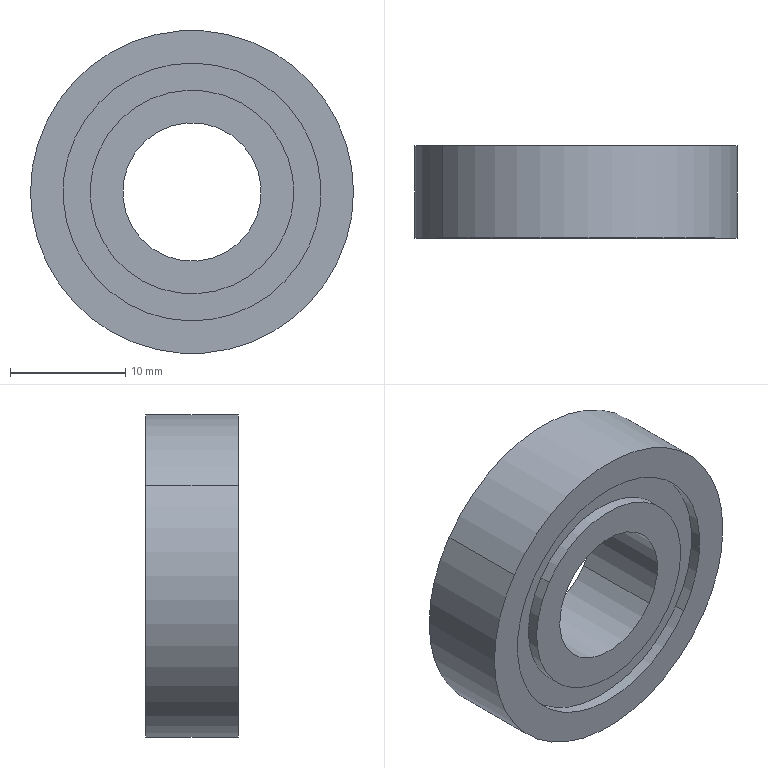Component | SolidWorks | UpperAxis-1_UpperSlideBearing-1 | 1 solid | 18 faces | box 28 x 8 x 28 mm | volume 3727 mm3 | cylinder 12 | plane 6 | commonest cylinder face diameters 17.655 x4 22.345 x4 28 x2 12 x2
build123d program:
from build123d import *


with BuildPart() as part:
    # Sketch1 → Revolve1 (revolve)
    with BuildSketch(Plane(origin=(0, 0, 0), x_dir=(1, 0, 0), z_dir=(0, 1, 0)), mode=Mode.PRIVATE) as revolve1_sk:
        Polygon((4, 4), (6.827, 4), (6.827, 3), (9.173, 3), (9.173, 4), (12, 4), (12, -4), (9.173, -4), (9.173, -3), (6.827, -3), (6.827, -4), (4, -4), align=None)
    revolve(revolve1_sk.sketch.rotate(Axis((-2, 0, -4.4), (0, 0, 1)), 180), axis=Axis((-2, 0, -4.4), (0, 0, 1)))


solid = part.part

# Placed as in the assembly
solid = solid.moved(Location((-776.65, 378.568, -31.569), (90, 0, 0)))
STEP:
#1=COLOUR_RGB('',0.7922,0.8196,0.9333);
#2=FILL_AREA_STYLE_COLOUR('',#1);
#3=FILL_AREA_STYLE('',(#2));
#4=SURFACE_STYLE_FILL_AREA(#3);
#5=SURFACE_SIDE_STYLE('',(#4));
#6=SURFACE_STYLE_USAGE(.BOTH.,#5);
#7=PRESENTATION_STYLE_ASSIGNMENT((#6));
#8=CARTESIAN_POINT('',(-30.943,14.747,-1.047));
#9=VERTEX_POINT('',#8);
#10=CARTESIAN_POINT('',(-30.368,14.747,-1.439));
#11=VERTEX_POINT('',#10);
#12=CARTESIAN_POINT('',(-30.655,14.747,-1.243));
#13=DIRECTION('',(-0.,1.,0.));
#14=DIRECTION('',(-0.8265,0.,0.563));
#15=AXIS2_PLACEMENT_3D('',#12,#13,#14);
#16=CIRCLE('',#15,0.3475);
#17=EDGE_CURVE('',#9,#11,#16,.T.);
#18=ORIENTED_EDGE('',*,*,#17,.T.);
#19=CARTESIAN_POINT('',(-30.368,14.786,-1.439));
#20=VERTEX_POINT('',#19);
#21=CARTESIAN_POINT('',(-30.368,15.077,-1.439));
#22=DIRECTION('',(-0.,1.,0.));
#23=VECTOR('',#22,39.37);
#24=LINE('',#21,#23);
#25=EDGE_CURVE('',#11,#20,#24,.T.);
#26=ORIENTED_EDGE('',*,*,#25,.T.);
#27=CARTESIAN_POINT('',(-30.943,14.786,-1.047));
#28=VERTEX_POINT('',#27);
#29=CARTESIAN_POINT('',(-30.655,14.786,-1.243));
#30=DIRECTION('',(-0.,1.,0.));
#31=DIRECTION('',(-0.8265,0.,0.563));
#32=AXIS2_PLACEMENT_3D('',#29,#30,#31);
#33=CIRCLE('',#32,0.3475);
#34=EDGE_CURVE('',#28,#20,#33,.T.);
#35=ORIENTED_EDGE('',*,*,#34,.F.);
#36=CARTESIAN_POINT('',(-30.943,15.077,-1.047));
#37=DIRECTION('',(-0.,1.,0.));
#38=VECTOR('',#37,39.37);
#39=LINE('',#36,#38);
#40=EDGE_CURVE('',#9,#28,#39,.T.);
#41=ORIENTED_EDGE('',*,*,#40,.F.);
#42=EDGE_LOOP('',(#18,#26,#35,#41));
#43=FACE_OUTER_BOUND('',#42,.T.);
#44=CARTESIAN_POINT('',(-30.655,15.077,-1.243));
#45=DIRECTION('',(-0.,1.,0.));
#46=DIRECTION('',(-0.8265,0.,0.563));
#47=AXIS2_PLACEMENT_3D('',#44,#45,#46);
#48=CYLINDRICAL_SURFACE('',#47,0.3475);
#49=ADVANCED_FACE('',(#43),#48,.T.);
#50=CARTESIAN_POINT('',(-30.292,14.747,-1.491));
#51=VERTEX_POINT('',#50);
#52=CARTESIAN_POINT('',(-31.019,14.747,-0.9953));
#53=VERTEX_POINT('',#52);
#54=CARTESIAN_POINT('',(-30.655,14.747,-1.243));
#55=DIRECTION('',(-0.,1.,0.));
#56=DIRECTION('',(-0.8265,0.,0.563));
#57=AXIS2_PLACEMENT_3D('',#54,#55,#56);
#58=CIRCLE('',#57,0.4399);
#59=EDGE_CURVE('',#51,#53,#58,.T.);
#60=ORIENTED_EDGE('',*,*,#59,.F.);
#61=CARTESIAN_POINT('',(-30.292,14.786,-1.491));
#62=VERTEX_POINT('',#61);
#63=CARTESIAN_POINT('',(-30.292,15.077,-1.491));
#64=DIRECTION('',(-0.,1.,0.));
#65=VECTOR('',#64,39.37);
#66=LINE('',#63,#65);
#67=EDGE_CURVE('',#51,#62,#66,.T.);
#68=ORIENTED_EDGE('',*,*,#67,.T.);
#69=CARTESIAN_POINT('',(-31.019,14.786,-0.9953));
#70=VERTEX_POINT('',#69);
#71=CARTESIAN_POINT('',(-30.655,14.786,-1.243));
#72=DIRECTION('',(-0.,1.,0.));
#73=DIRECTION('',(-0.8265,0.,0.563));
#74=AXIS2_PLACEMENT_3D('',#71,#72,#73);
#75=CIRCLE('',#74,0.4399);
#76=EDGE_CURVE('',#62,#70,#75,.T.);
#77=ORIENTED_EDGE('',*,*,#76,.T.);
#78=CARTESIAN_POINT('',(-31.019,15.077,-0.9953));
#79=DIRECTION('',(-0.,1.,0.));
#80=VECTOR('',#79,39.37);
#81=LINE('',#78,#80);
#82=EDGE_CURVE('',#53,#70,#81,.T.);
#83=ORIENTED_EDGE('',*,*,#82,.F.);
#84=EDGE_LOOP('',(#60,#68,#77,#83));
#85=FACE_OUTER_BOUND('',#84,.T.);
#86=CARTESIAN_POINT('',(-30.655,15.077,-1.243));
#87=DIRECTION('',(-0.,1.,0.));
#88=DIRECTION('',(-0.8265,0.,0.563));
#89=AXIS2_PLACEMENT_3D('',#86,#87,#88);
#90=CYLINDRICAL_SURFACE('',#89,0.4399);
#91=ADVANCED_FACE('',(#85),#90,.F.);
#92=CARTESIAN_POINT('',(-31.111,14.747,-0.9326));
#93=VERTEX_POINT('',#92);
#94=CARTESIAN_POINT('',(-30.2,14.747,-1.553));
#95=VERTEX_POINT('',#94);
#96=CARTESIAN_POINT('',(-30.655,14.747,-1.243));
#97=DIRECTION('',(-0.,1.,0.));
#98=DIRECTION('',(-0.8265,0.,0.563));
#99=AXIS2_PLACEMENT_3D('',#96,#97,#98);
#100=CIRCLE('',#99,0.5512);
#101=EDGE_CURVE('',#93,#95,#100,.T.);
#102=ORIENTED_EDGE('',*,*,#101,.T.);
#103=CARTESIAN_POINT('',(-30.2,15.062,-1.553));
#104=VERTEX_POINT('',#103);
#105=CARTESIAN_POINT('',(-30.2,15.077,-1.553));
#106=DIRECTION('',(-0.,1.,0.));
#107=VECTOR('',#106,39.37);
#108=LINE('',#105,#107);
#109=EDGE_CURVE('',#95,#104,#108,.T.);
#110=ORIENTED_EDGE('',*,*,#109,.T.);
#111=CARTESIAN_POINT('',(-31.111,15.062,-0.9326));
#112=VERTEX_POINT('',#111);
#113=CARTESIAN_POINT('',(-30.655,15.062,-1.243));
#114=DIRECTION('',(-0.,1.,0.));
#115=DIRECTION('',(-0.8265,0.,0.563));
#116=AXIS2_PLACEMENT_3D('',#113,#114,#115);
#117=CIRCLE('',#116,0.5512);
#118=EDGE_CURVE('',#112,#104,#117,.T.);
#119=ORIENTED_EDGE('',*,*,#118,.F.);
#120=CARTESIAN_POINT('',(-31.111,15.077,-0.9326));
#121=DIRECTION('',(-0.,1.,0.));
#122=VECTOR('',#121,39.37);
#123=LINE('',#120,#122);
#124=EDGE_CURVE('',#93,#112,#123,.T.);
#125=ORIENTED_EDGE('',*,*,#124,.F.);
#126=EDGE_LOOP('',(#102,#110,#119,#125));
#127=FACE_OUTER_BOUND('',#126,.T.);
#128=CARTESIAN_POINT('',(-30.655,15.077,-1.243));
#129=DIRECTION('',(-0.,1.,0.));
#130=DIRECTION('',(-0.8265,0.,0.563));
#131=AXIS2_PLACEMENT_3D('',#128,#129,#130);
#132=CYLINDRICAL_SURFACE('',#131,0.5512);
#133=ADVANCED_FACE('',(#127),#132,.T.);
#134=CARTESIAN_POINT('',(-30.292,15.022,-1.491));
#135=VERTEX_POINT('',#134);
#136=CARTESIAN_POINT('',(-31.019,15.022,-0.9953));
#137=VERTEX_POINT('',#136);
#138=CARTESIAN_POINT('',(-30.655,15.022,-1.243));
#139=DIRECTION('',(-0.,1.,0.));
#140=DIRECTION('',(-0.8265,0.,0.563));
#141=AXIS2_PLACEMENT_3D('',#138,#139,#140);
#142=CIRCLE('',#141,0.4399);
#143=EDGE_CURVE('',#135,#137,#142,.T.);
#144=ORIENTED_EDGE('',*,*,#143,.F.);
#145=CARTESIAN_POINT('',(-30.292,15.062,-1.491));
#146=VERTEX_POINT('',#145);
#147=CARTESIAN_POINT('',(-30.292,15.077,-1.491));
#148=DIRECTION('',(-0.,1.,0.));
#149=VECTOR('',#148,39.37);
#150=LINE('',#147,#149);
#151=EDGE_CURVE('',#135,#146,#150,.T.);
#152=ORIENTED_EDGE('',*,*,#151,.T.);
#153=CARTESIAN_POINT('',(-31.019,15.062,-0.9953));
#154=VERTEX_POINT('',#153);
#155=CARTESIAN_POINT('',(-30.655,15.062,-1.243));
#156=DIRECTION('',(-0.,1.,0.));
#157=DIRECTION('',(-0.8265,0.,0.563));
#158=AXIS2_PLACEMENT_3D('',#155,#156,#157);
#159=CIRCLE('',#158,0.4399);
#160=EDGE_CURVE('',#146,#154,#159,.T.);
#161=ORIENTED_EDGE('',*,*,#160,.T.);
#162=CARTESIAN_POINT('',(-31.019,15.077,-0.9953));
#163=DIRECTION('',(-0.,1.,0.));
#164=VECTOR('',#163,39.37);
#165=LINE('',#162,#164);
#166=EDGE_CURVE('',#137,#154,#165,.T.);
#167=ORIENTED_EDGE('',*,*,#166,.F.);
#168=EDGE_LOOP('',(#144,#152,#161,#167));
#169=FACE_OUTER_BOUND('',#168,.T.);
#170=CARTESIAN_POINT('',(-30.655,15.077,-1.243));
#171=DIRECTION('',(-0.,1.,0.));
#172=DIRECTION('',(-0.8265,0.,0.563));
#173=AXIS2_PLACEMENT_3D('',#170,#171,#172);
#174=CYLINDRICAL_SURFACE('',#173,0.4399);
#175=ADVANCED_FACE('',(#169),#174,.F.);
#176=CARTESIAN_POINT('',(-30.943,15.022,-1.047));
#177=VERTEX_POINT('',#176);
#178=CARTESIAN_POINT('',(-30.368,15.022,-1.439));
#179=VERTEX_POINT('',#178);
#180=CARTESIAN_POINT('',(-30.655,15.022,-1.243));
#181=DIRECTION('',(-0.,1.,0.));
#182=DIRECTION('',(-0.8265,0.,0.563));
#183=AXIS2_PLACEMENT_3D('',#180,#181,#182);
#184=CIRCLE('',#183,0.3475);
#185=EDGE_CURVE('',#177,#179,#184,.T.);
#186=ORIENTED_EDGE('',*,*,#185,.T.);
#187=CARTESIAN_POINT('',(-30.368,15.062,-1.439));
#188=VERTEX_POINT('',#187);
#189=CARTESIAN_POINT('',(-30.368,15.077,-1.439));
#190=DIRECTION('',(-0.,1.,0.));
#191=VECTOR('',#190,39.37);
#192=LINE('',#189,#191);
#193=EDGE_CURVE('',#179,#188,#192,.T.);
#194=ORIENTED_EDGE('',*,*,#193,.T.);
#195=CARTESIAN_POINT('',(-30.943,15.062,-1.047));
#196=VERTEX_POINT('',#195);
#197=CARTESIAN_POINT('',(-30.655,15.062,-1.243));
#198=DIRECTION('',(-0.,1.,0.));
#199=DIRECTION('',(-0.8265,0.,0.563));
#200=AXIS2_PLACEMENT_3D('',#197,#198,#199);
#201=CIRCLE('',#200,0.3475);
#202=EDGE_CURVE('',#196,#188,#201,.T.);
#203=ORIENTED_EDGE('',*,*,#202,.F.);
#204=CARTESIAN_POINT('',(-30.943,15.077,-1.047));
#205=DIRECTION('',(-0.,1.,0.));
#206=VECTOR('',#205,39.37);
#207=LINE('',#204,#206);
#208=EDGE_CURVE('',#177,#196,#207,.T.);
#209=ORIENTED_EDGE('',*,*,#208,.F.);
#210=EDGE_LOOP('',(#186,#194,#203,#209));
#211=FACE_OUTER_BOUND('',#210,.T.);
#212=CARTESIAN_POINT('',(-30.655,15.077,-1.243));
#213=DIRECTION('',(-0.,1.,0.));
#214=DIRECTION('',(-0.8265,0.,0.563));
#215=AXIS2_PLACEMENT_3D('',#212,#213,#214);
#216=CYLINDRICAL_SURFACE('',#215,0.3475);
#217=ADVANCED_FACE('',(#211),#216,.T.);
#218=CARTESIAN_POINT('',(-30.46,14.747,-1.376));
#219=VERTEX_POINT('',#218);
#220=CARTESIAN_POINT('',(-30.851,14.747,-1.11));
#221=VERTEX_POINT('',#220);
#222=CARTESIAN_POINT('',(-30.655,14.747,-1.243));
#223=DIRECTION('',(-0.,1.,0.));
#224=DIRECTION('',(-0.8265,0.,0.563));
#225=AXIS2_PLACEMENT_3D('',#222,#223,#224);
#226=CIRCLE('',#225,0.2362);
#227=EDGE_CURVE('',#219,#221,#226,.T.);
#228=ORIENTED_EDGE('',*,*,#227,.F.);
#229=CARTESIAN_POINT('',(-30.46,15.062,-1.376));
#230=VERTEX_POINT('',#229);
#231=CARTESIAN_POINT('',(-30.46,15.077,-1.376));
#232=DIRECTION('',(-0.,1.,0.));
#233=VECTOR('',#232,39.37);
#234=LINE('',#231,#233);
#235=EDGE_CURVE('',#219,#230,#234,.T.);
#236=ORIENTED_EDGE('',*,*,#235,.T.);
#237=CARTESIAN_POINT('',(-30.851,15.062,-1.11));
#238=VERTEX_POINT('',#237);
#239=CARTESIAN_POINT('',(-30.655,15.062,-1.243));
#240=DIRECTION('',(-0.,1.,0.));
#241=DIRECTION('',(-0.8265,0.,0.563));
#242=AXIS2_PLACEMENT_3D('',#239,#240,#241);
#243=CIRCLE('',#242,0.2362);
#244=EDGE_CURVE('',#230,#238,#243,.T.);
#245=ORIENTED_EDGE('',*,*,#244,.T.);
#246=CARTESIAN_POINT('',(-30.851,15.077,-1.11));
#247=DIRECTION('',(-0.,1.,0.));
#248=VECTOR('',#247,39.37);
#249=LINE('',#246,#248);
#250=EDGE_CURVE('',#221,#238,#249,.T.);
#251=ORIENTED_EDGE('',*,*,#250,.F.);
#252=EDGE_LOOP('',(#228,#236,#245,#251));
#253=FACE_OUTER_BOUND('',#252,.T.);
#254=CARTESIAN_POINT('',(-30.655,15.077,-1.243));
#255=DIRECTION('',(-0.,1.,0.));
#256=DIRECTION('',(-0.8265,0.,0.563));
#257=AXIS2_PLACEMENT_3D('',#254,#255,#256);
#258=CYLINDRICAL_SURFACE('',#257,0.2362);
#259=ADVANCED_FACE('',(#253),#258,.F.);
#260=ORIENTED_EDGE('',*,*,#235,.F.);
#261=CARTESIAN_POINT('',(-30.655,14.747,-1.243));
#262=DIRECTION('',(-0.,1.,0.));
#263=DIRECTION('',(-0.8265,0.,0.563));
#264=AXIS2_PLACEMENT_3D('',#261,#262,#263);
#265=CIRCLE('',#264,0.2362);
#266=EDGE_CURVE('',#221,#219,#265,.T.);
#267=ORIENTED_EDGE('',*,*,#266,.F.);
#268=ORIENTED_EDGE('',*,*,#250,.T.);
#269=CARTESIAN_POINT('',(-30.655,15.062,-1.243));
#270=DIRECTION('',(-0.,1.,0.));
#271=DIRECTION('',(-0.8265,0.,0.563));
#272=AXIS2_PLACEMENT_3D('',#269,#270,#271);
#273=CIRCLE('',#272,0.2362);
#274=EDGE_CURVE('',#238,#230,#273,.T.);
#275=ORIENTED_EDGE('',*,*,#274,.T.);
#276=EDGE_LOOP('',(#260,#267,#268,#275));
#277=FACE_OUTER_BOUND('',#276,.T.);
#278=CARTESIAN_POINT('',(-30.655,15.077,-1.243));
#279=DIRECTION('',(-0.,1.,0.));
#280=DIRECTION('',(-0.8265,0.,0.563));
#281=AXIS2_PLACEMENT_3D('',#278,#279,#280);
#282=CYLINDRICAL_SURFACE('',#281,0.2362);
#283=ADVANCED_FACE('',(#277),#282,.F.);
#284=ORIENTED_EDGE('',*,*,#274,.F.);
#285=ORIENTED_EDGE('',*,*,#244,.F.);
#286=EDGE_LOOP('',(#284,#285));
#287=FACE_BOUND('',#286,.T.);
#288=ORIENTED_EDGE('',*,*,#202,.T.);
#289=CARTESIAN_POINT('',(-30.655,15.062,-1.243));
#290=DIRECTION('',(-0.,1.,0.));
#291=DIRECTION('',(-0.8265,0.,0.563));
#292=AXIS2_PLACEMENT_3D('',#289,#290,#291);
#293=CIRCLE('',#292,0.3475);
#294=EDGE_CURVE('',#188,#196,#293,.T.);
#295=ORIENTED_EDGE('',*,*,#294,.T.);
#296=EDGE_LOOP('',(#288,#295));
#297=FACE_OUTER_BOUND('',#296,.T.);
#298=CARTESIAN_POINT('',(-30.46,15.062,-1.376));
#299=DIRECTION('',(0.,-1.,-0.));
#300=DIRECTION('',(0.8265,0.,-0.563));
#301=AXIS2_PLACEMENT_3D('',#298,#299,#300);
#302=PLANE('',#301);
#303=ADVANCED_FACE('',(#287,#297),#302,.F.);
#304=ORIENTED_EDGE('',*,*,#193,.F.);
#305=CARTESIAN_POINT('',(-30.655,15.022,-1.243));
#306=DIRECTION('',(-0.,1.,0.));
#307=DIRECTION('',(-0.8265,0.,0.563));
#308=AXIS2_PLACEMENT_3D('',#305,#306,#307);
#309=CIRCLE('',#308,0.3475);
#310=EDGE_CURVE('',#179,#177,#309,.T.);
#311=ORIENTED_EDGE('',*,*,#310,.T.);
#312=ORIENTED_EDGE('',*,*,#208,.T.);
#313=ORIENTED_EDGE('',*,*,#294,.F.);
#314=EDGE_LOOP('',(#304,#311,#312,#313));
#315=FACE_OUTER_BOUND('',#314,.T.);
#316=CARTESIAN_POINT('',(-30.655,15.077,-1.243));
#317=DIRECTION('',(-0.,1.,0.));
#318=DIRECTION('',(-0.8265,0.,0.563));
#319=AXIS2_PLACEMENT_3D('',#316,#317,#318);
#320=CYLINDRICAL_SURFACE('',#319,0.3475);
#321=ADVANCED_FACE('',(#315),#320,.T.);
#322=ORIENTED_EDGE('',*,*,#185,.F.);
#323=ORIENTED_EDGE('',*,*,#310,.F.);
#324=EDGE_LOOP('',(#322,#323));
#325=FACE_BOUND('',#324,.T.);
#326=CARTESIAN_POINT('',(-30.655,15.022,-1.243));
#327=DIRECTION('',(-0.,1.,0.));
#328=DIRECTION('',(-0.8265,0.,0.563));
#329=AXIS2_PLACEMENT_3D('',#326,#327,#328);
#330=CIRCLE('',#329,0.4399);
#331=EDGE_CURVE('',#137,#135,#330,.T.);
#332=ORIENTED_EDGE('',*,*,#331,.T.);
#333=ORIENTED_EDGE('',*,*,#143,.T.);
#334=EDGE_LOOP('',(#332,#333));
#335=FACE_OUTER_BOUND('',#334,.T.);
#336=CARTESIAN_POINT('',(-30.292,15.022,-1.491));
#337=DIRECTION('',(0.,-1.,-0.));
#338=DIRECTION('',(0.8265,0.,-0.563));
#339=AXIS2_PLACEMENT_3D('',#336,#337,#338);
#340=PLANE('',#339);
#341=ADVANCED_FACE('',(#325,#335),#340,.F.);
#342=ORIENTED_EDGE('',*,*,#151,.F.);
#343=ORIENTED_EDGE('',*,*,#331,.F.);
#344=ORIENTED_EDGE('',*,*,#166,.T.);
#345=CARTESIAN_POINT('',(-30.655,15.062,-1.243));
#346=DIRECTION('',(-0.,1.,0.));
#347=DIRECTION('',(-0.8265,0.,0.563));
#348=AXIS2_PLACEMENT_3D('',#345,#346,#347);
#349=CIRCLE('',#348,0.4399);
#350=EDGE_CURVE('',#154,#146,#349,.T.);
#351=ORIENTED_EDGE('',*,*,#350,.T.);
#352=EDGE_LOOP('',(#342,#343,#344,#351));
#353=FACE_OUTER_BOUND('',#352,.T.);
#354=CARTESIAN_POINT('',(-30.655,15.077,-1.243));
#355=DIRECTION('',(-0.,1.,0.));
#356=DIRECTION('',(-0.8265,0.,0.563));
#357=AXIS2_PLACEMENT_3D('',#354,#355,#356);
#358=CYLINDRICAL_SURFACE('',#357,0.4399);
#359=ADVANCED_FACE('',(#353),#358,.F.);
#360=ORIENTED_EDGE('',*,*,#350,.F.);
#361=ORIENTED_EDGE('',*,*,#160,.F.);
#362=EDGE_LOOP('',(#360,#361));
#363=FACE_BOUND('',#362,.T.);
#364=ORIENTED_EDGE('',*,*,#118,.T.);
#365=CARTESIAN_POINT('',(-30.655,15.062,-1.243));
#366=DIRECTION('',(-0.,1.,0.));
#367=DIRECTION('',(-0.8265,0.,0.563));
#368=AXIS2_PLACEMENT_3D('',#365,#366,#367);
#369=CIRCLE('',#368,0.5512);
#370=EDGE_CURVE('',#104,#112,#369,.T.);
#371=ORIENTED_EDGE('',*,*,#370,.T.);
#372=EDGE_LOOP('',(#364,#371));
#373=FACE_OUTER_BOUND('',#372,.T.);
#374=CARTESIAN_POINT('',(-30.292,15.062,-1.491));
#375=DIRECTION('',(0.,-1.,-0.));
#376=DIRECTION('',(0.8265,0.,-0.563));
#377=AXIS2_PLACEMENT_3D('',#374,#375,#376);
#378=PLANE('',#377);
#379=ADVANCED_FACE('',(#363,#373),#378,.F.);
#380=ORIENTED_EDGE('',*,*,#109,.F.);
#381=CARTESIAN_POINT('',(-30.655,14.747,-1.243));
#382=DIRECTION('',(-0.,1.,0.));
#383=DIRECTION('',(-0.8265,0.,0.563));
#384=AXIS2_PLACEMENT_3D('',#381,#382,#383);
#385=CIRCLE('',#384,0.5512);
#386=EDGE_CURVE('',#95,#93,#385,.T.);
#387=ORIENTED_EDGE('',*,*,#386,.T.);
#388=ORIENTED_EDGE('',*,*,#124,.T.);
#389=ORIENTED_EDGE('',*,*,#370,.F.);
#390=EDGE_LOOP('',(#380,#387,#388,#389));
#391=FACE_OUTER_BOUND('',#390,.T.);
#392=CARTESIAN_POINT('',(-30.655,15.077,-1.243));
#393=DIRECTION('',(-0.,1.,0.));
#394=DIRECTION('',(-0.8265,0.,0.563));
#395=AXIS2_PLACEMENT_3D('',#392,#393,#394);
#396=CYLINDRICAL_SURFACE('',#395,0.5512);
#397=ADVANCED_FACE('',(#391),#396,.T.);
#398=ORIENTED_EDGE('',*,*,#101,.F.);
#399=ORIENTED_EDGE('',*,*,#386,.F.);
#400=EDGE_LOOP('',(#398,#399));
#401=FACE_OUTER_BOUND('',#400,.T.);
#402=CARTESIAN_POINT('',(-30.655,14.747,-1.243));
#403=DIRECTION('',(-0.,1.,0.));
#404=DIRECTION('',(-0.8265,0.,0.563));
#405=AXIS2_PLACEMENT_3D('',#402,#403,#404);
#406=CIRCLE('',#405,0.4399);
#407=EDGE_CURVE('',#53,#51,#406,.T.);
#408=ORIENTED_EDGE('',*,*,#407,.T.);
#409=ORIENTED_EDGE('',*,*,#59,.T.);
#410=EDGE_LOOP('',(#408,#409));
#411=FACE_BOUND('',#410,.T.);
#412=CARTESIAN_POINT('',(-30.2,14.747,-1.553));
#413=DIRECTION('',(-0.,1.,0.));
#414=DIRECTION('',(-0.8265,-0.,0.563));
#415=AXIS2_PLACEMENT_3D('',#412,#413,#414);
#416=PLANE('',#415);
#417=ADVANCED_FACE('',(#401,#411),#416,.F.);
#418=ORIENTED_EDGE('',*,*,#67,.F.);
#419=ORIENTED_EDGE('',*,*,#407,.F.);
#420=ORIENTED_EDGE('',*,*,#82,.T.);
#421=CARTESIAN_POINT('',(-30.655,14.786,-1.243));
#422=DIRECTION('',(-0.,1.,0.));
#423=DIRECTION('',(-0.8265,0.,0.563));
#424=AXIS2_PLACEMENT_3D('',#421,#422,#423);
#425=CIRCLE('',#424,0.4399);
#426=EDGE_CURVE('',#70,#62,#425,.T.);
#427=ORIENTED_EDGE('',*,*,#426,.T.);
#428=EDGE_LOOP('',(#418,#419,#420,#427));
#429=FACE_OUTER_BOUND('',#428,.T.);
#430=CARTESIAN_POINT('',(-30.655,15.077,-1.243));
#431=DIRECTION('',(-0.,1.,0.));
#432=DIRECTION('',(-0.8265,0.,0.563));
#433=AXIS2_PLACEMENT_3D('',#430,#431,#432);
#434=CYLINDRICAL_SURFACE('',#433,0.4399);
#435=ADVANCED_FACE('',(#429),#434,.F.);
#436=ORIENTED_EDGE('',*,*,#426,.F.);
#437=ORIENTED_EDGE('',*,*,#76,.F.);
#438=EDGE_LOOP('',(#436,#437));
#439=FACE_OUTER_BOUND('',#438,.T.);
#440=ORIENTED_EDGE('',*,*,#34,.T.);
#441=CARTESIAN_POINT('',(-30.655,14.786,-1.243));
#442=DIRECTION('',(-0.,1.,0.));
#443=DIRECTION('',(-0.8265,0.,0.563));
#444=AXIS2_PLACEMENT_3D('',#441,#442,#443);
#445=CIRCLE('',#444,0.3475);
#446=EDGE_CURVE('',#20,#28,#445,.T.);
#447=ORIENTED_EDGE('',*,*,#446,.T.);
#448=EDGE_LOOP('',(#440,#447));
#449=FACE_BOUND('',#448,.T.);
#450=CARTESIAN_POINT('',(-30.292,14.786,-1.491));
#451=DIRECTION('',(-0.,1.,0.));
#452=DIRECTION('',(-0.8265,-0.,0.563));
#453=AXIS2_PLACEMENT_3D('',#450,#451,#452);
#454=PLANE('',#453);
#455=ADVANCED_FACE('',(#439,#449),#454,.F.);
#456=ORIENTED_EDGE('',*,*,#25,.F.);
#457=CARTESIAN_POINT('',(-30.655,14.747,-1.243));
#458=DIRECTION('',(-0.,1.,0.));
#459=DIRECTION('',(-0.8265,0.,0.563));
#460=AXIS2_PLACEMENT_3D('',#457,#458,#459);
#461=CIRCLE('',#460,0.3475);
#462=EDGE_CURVE('',#11,#9,#461,.T.);
#463=ORIENTED_EDGE('',*,*,#462,.T.);
#464=ORIENTED_EDGE('',*,*,#40,.T.);
#465=ORIENTED_EDGE('',*,*,#446,.F.);
#466=EDGE_LOOP('',(#456,#463,#464,#465));
#467=FACE_OUTER_BOUND('',#466,.T.);
#468=CARTESIAN_POINT('',(-30.655,15.077,-1.243));
#469=DIRECTION('',(-0.,1.,0.));
#470=DIRECTION('',(-0.8265,0.,0.563));
#471=AXIS2_PLACEMENT_3D('',#468,#469,#470);
#472=CYLINDRICAL_SURFACE('',#471,0.3475);
#473=ADVANCED_FACE('',(#467),#472,.T.);
#474=ORIENTED_EDGE('',*,*,#17,.F.);
#475=ORIENTED_EDGE('',*,*,#462,.F.);
#476=EDGE_LOOP('',(#474,#475));
#477=FACE_OUTER_BOUND('',#476,.T.);
#478=ORIENTED_EDGE('',*,*,#266,.T.);
#479=ORIENTED_EDGE('',*,*,#227,.T.);
#480=EDGE_LOOP('',(#478,#479));
#481=FACE_BOUND('',#480,.T.);
#482=CARTESIAN_POINT('',(-30.368,14.747,-1.439));
#483=DIRECTION('',(-0.,1.,0.));
#484=DIRECTION('',(-0.8265,-0.,0.563));
#485=AXIS2_PLACEMENT_3D('',#482,#483,#484);
#486=PLANE('',#485);
#487=ADVANCED_FACE('',(#477,#481),#486,.F.);
#488=CLOSED_SHELL('',(#49,#91,#133,#175,#217,#259,#283,#303,#321,#341,#359,#379,#397,#417,#435,#455,#473,#487));
#489=MANIFOLD_SOLID_BREP('',#488);
#490=STYLED_ITEM('',(#7),#489);
#491=PRESENTATION_LAYER_ASSIGNMENT('','',(#490));
#492=(LENGTH_UNIT()NAMED_UNIT(*)SI_UNIT($,.METRE.));
#493=LENGTH_MEASURE_WITH_UNIT(LENGTH_MEASURE(0.0254),#492);
#494=DIMENSIONAL_EXPONENTS(1.,0.,0.,0.,0.,0.,0.);
#495=(CONVERSION_BASED_UNIT('',#493)LENGTH_UNIT()NAMED_UNIT(#494));
#496=UNCERTAINTY_MEASURE_WITH_UNIT(LENGTH_MEASURE(0.00001),#495,'','');
#497=(NAMED_UNIT(*)PLANE_ANGLE_UNIT()SI_UNIT($,.RADIAN.));
#498=(NAMED_UNIT(*)SI_UNIT($,.STERADIAN.)SOLID_ANGLE_UNIT());
#499=(GEOMETRIC_REPRESENTATION_CONTEXT(3)GLOBAL_UNCERTAINTY_ASSIGNED_CONTEXT((#496))GLOBAL_UNIT_ASSIGNED_CONTEXT((#495,#497,#498))REPRESENTATION_CONTEXT('',''));
#500=MECHANICAL_DESIGN_GEOMETRIC_PRESENTATION_REPRESENTATION('',(#490),#499);
#501=CARTESIAN_POINT('',(0.,0.,0.));
#502=DIRECTION('',(0.,0.,1.));
#503=DIRECTION('',(1.,0.,0.));
#504=AXIS2_PLACEMENT_3D('',#501,#502,#503);
#505=(LENGTH_UNIT()NAMED_UNIT(*)SI_UNIT($,.METRE.));
#506=LENGTH_MEASURE_WITH_UNIT(LENGTH_MEASURE(0.0254),#505);
#507=DIMENSIONAL_EXPONENTS(1.,0.,0.,0.,0.,0.,0.);
#508=(CONVERSION_BASED_UNIT('',#506)LENGTH_UNIT()NAMED_UNIT(#507));
#509=UNCERTAINTY_MEASURE_WITH_UNIT(LENGTH_MEASURE(0.00001),#508,'','');
#510=(NAMED_UNIT(*)PLANE_ANGLE_UNIT()SI_UNIT($,.RADIAN.));
#511=(NAMED_UNIT(*)SI_UNIT($,.STERADIAN.)SOLID_ANGLE_UNIT());
#512=(GEOMETRIC_REPRESENTATION_CONTEXT(3)GLOBAL_UNCERTAINTY_ASSIGNED_CONTEXT((#509))GLOBAL_UNIT_ASSIGNED_CONTEXT((#508,#510,#511))REPRESENTATION_CONTEXT('',''));
#513=ADVANCED_BREP_SHAPE_REPRESENTATION('',(#489,#504),#512);